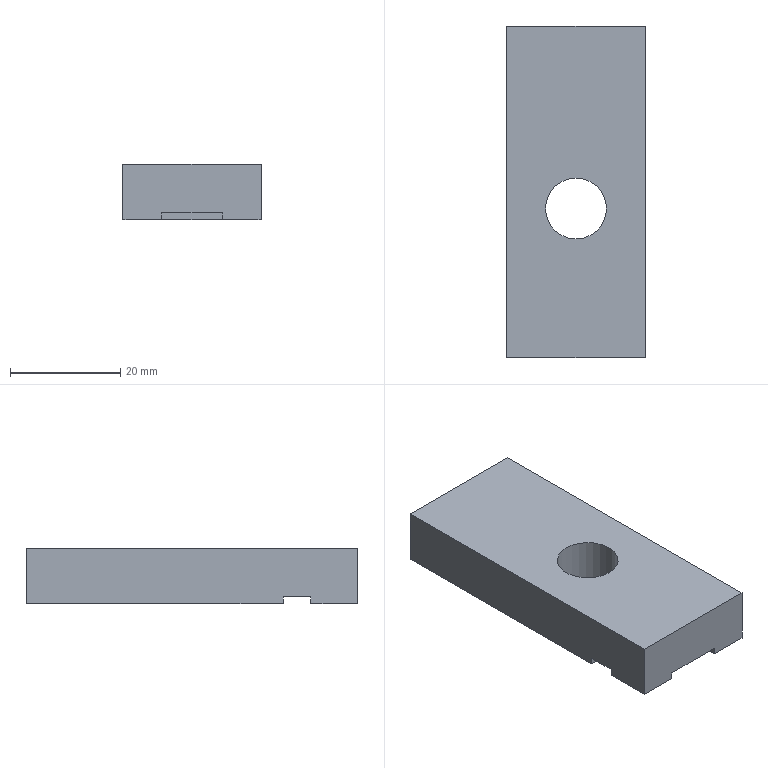Component | NX | CLAMP_PLATE | 1 solid | 19 faces | volume 13051 mm3 | plane 17 | cylinder 2 | commonest cylinder face diameters 11 x1 25 x1